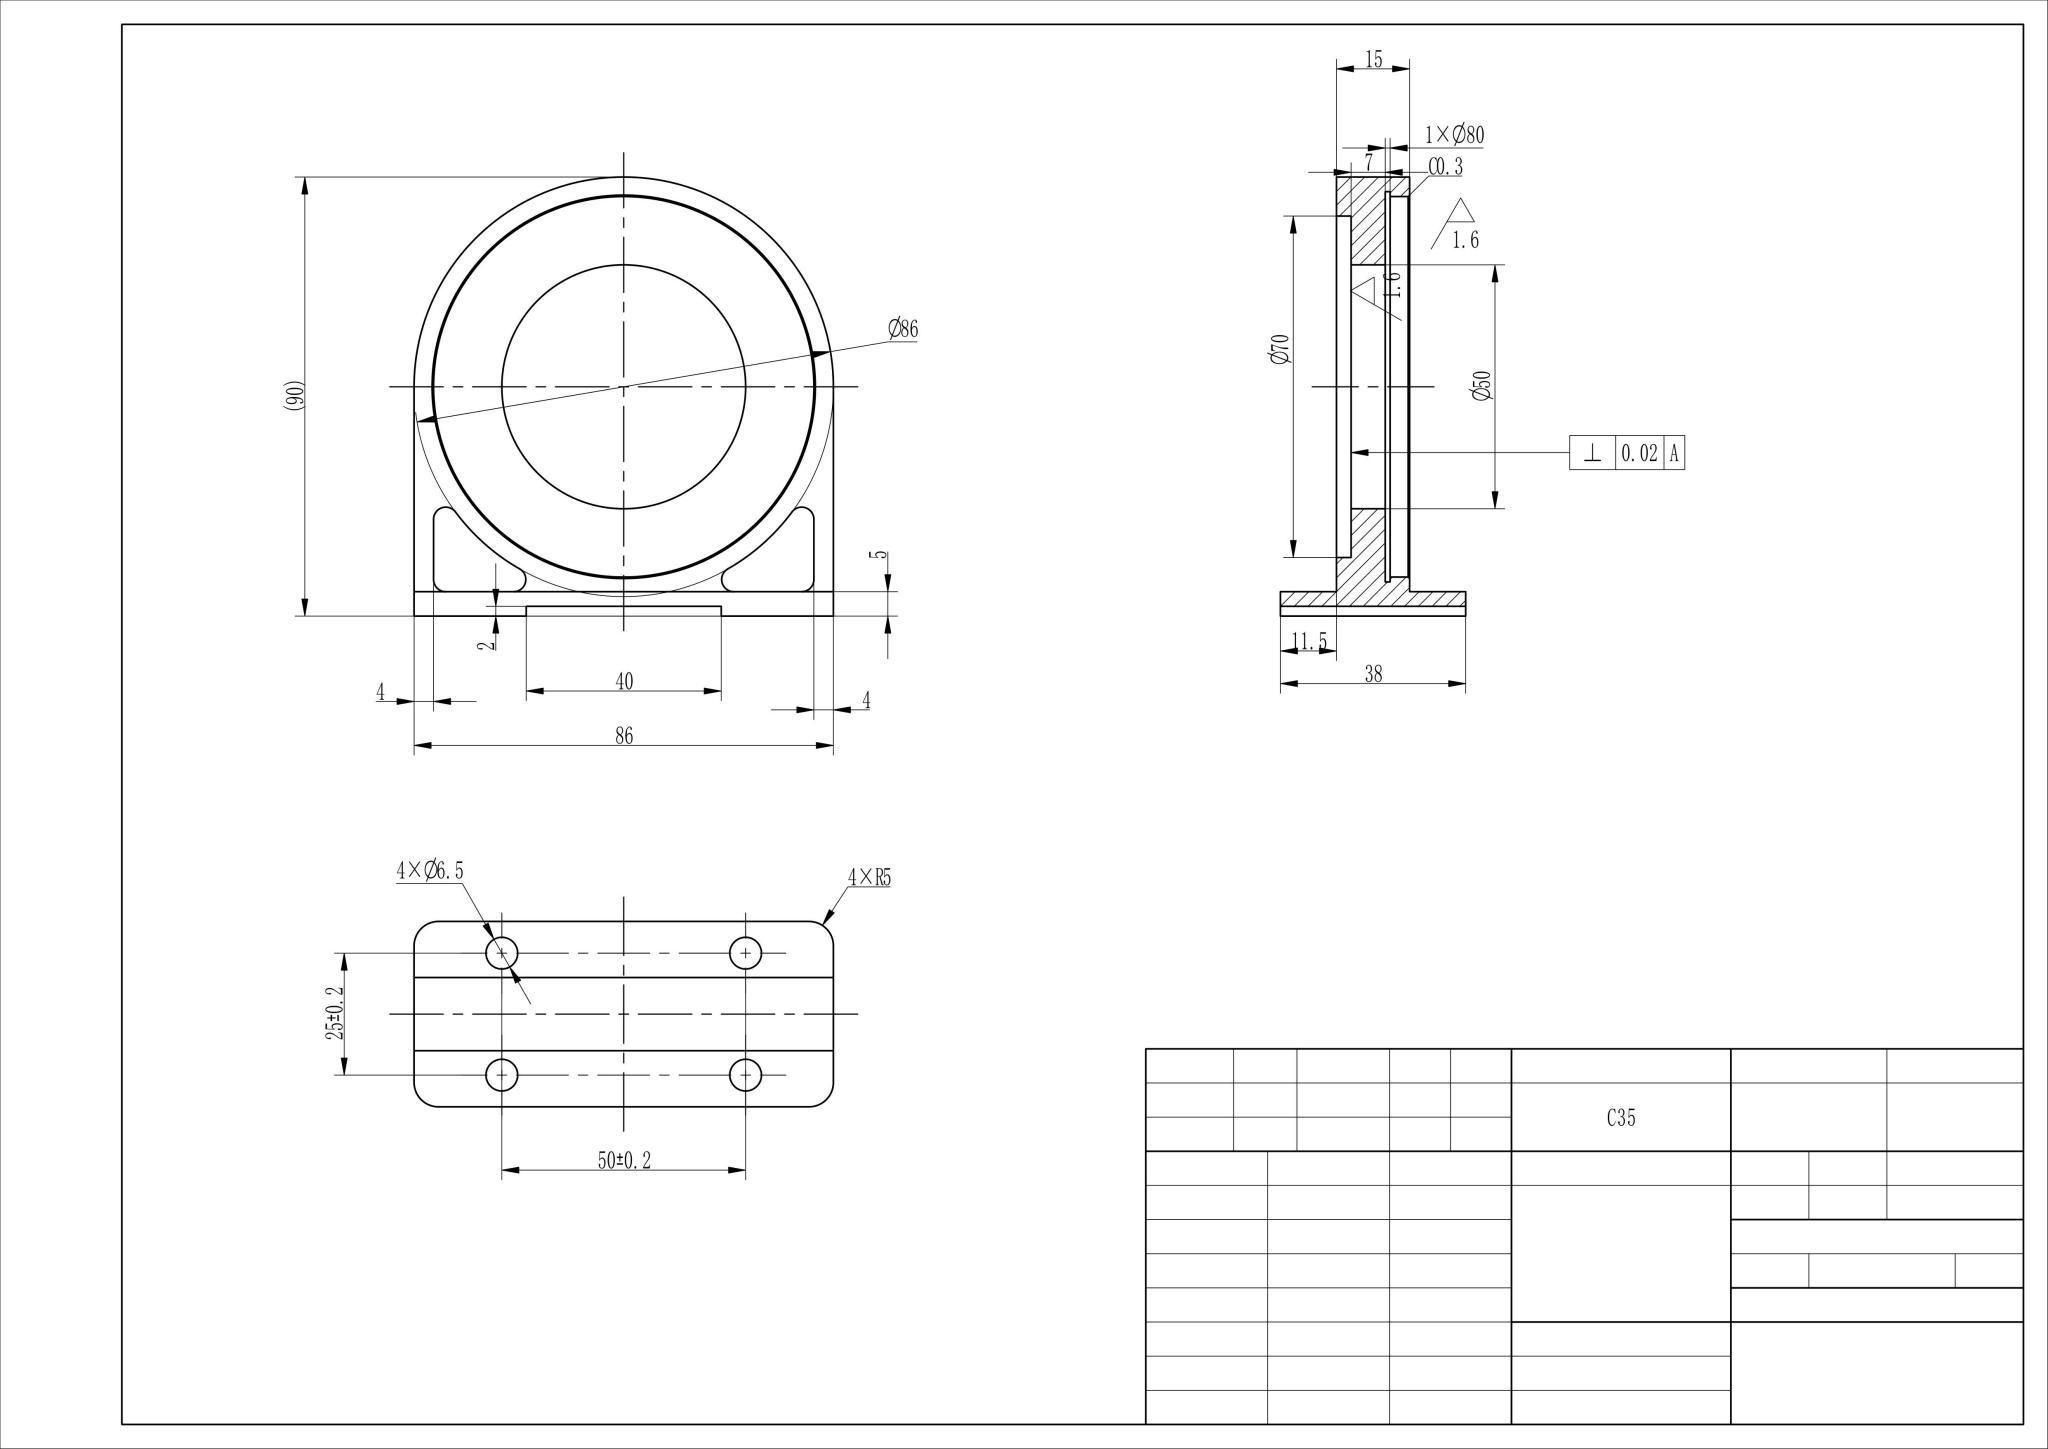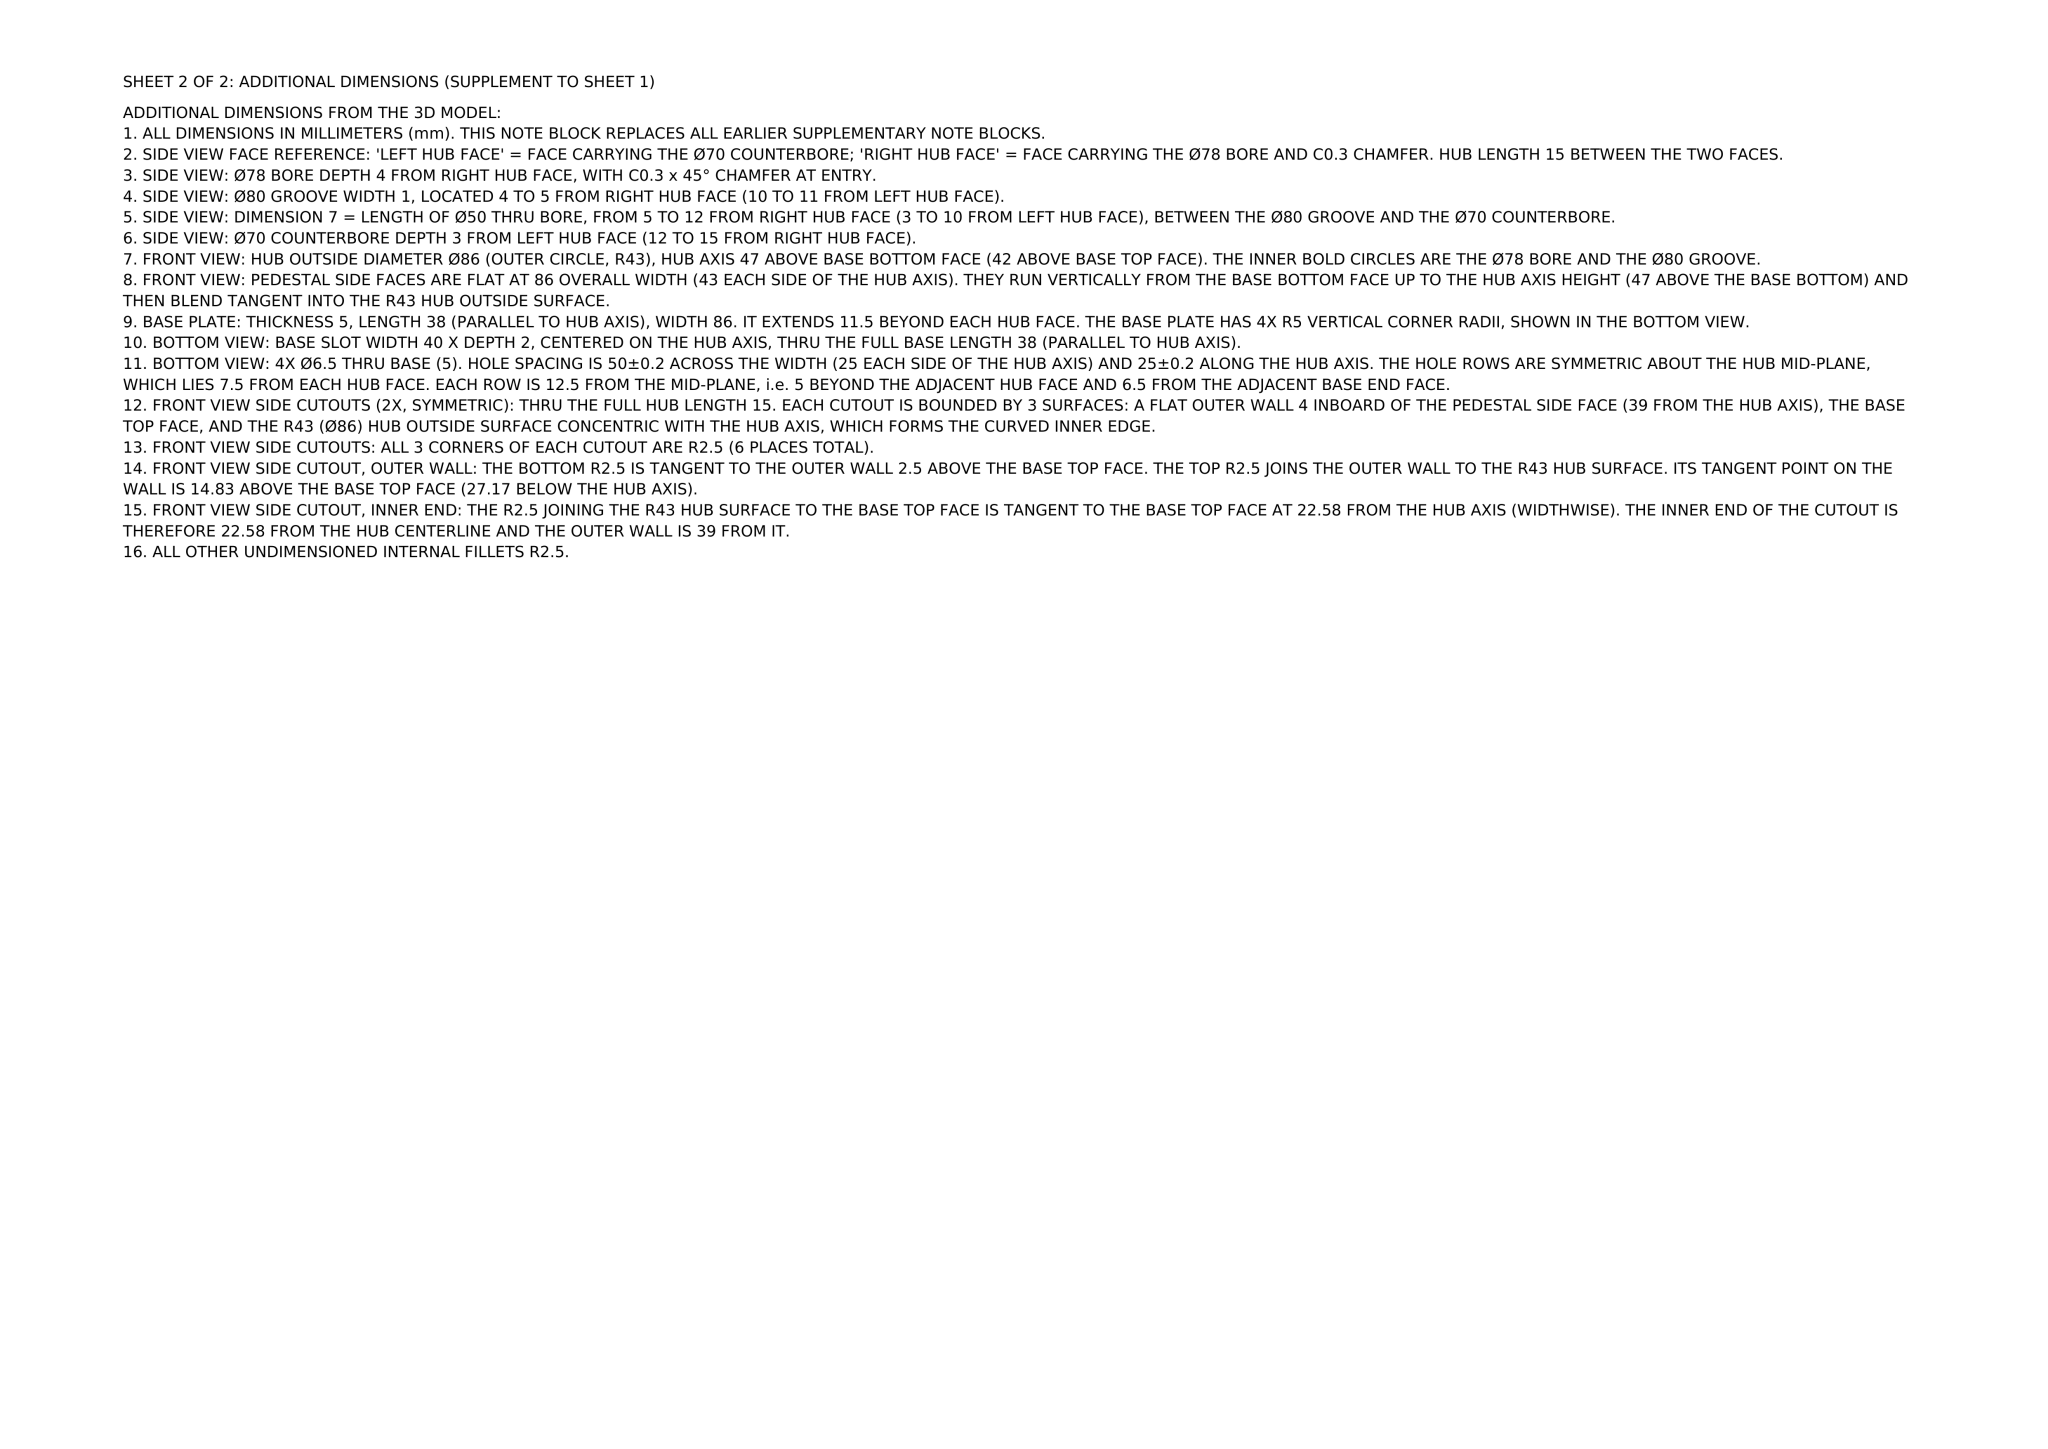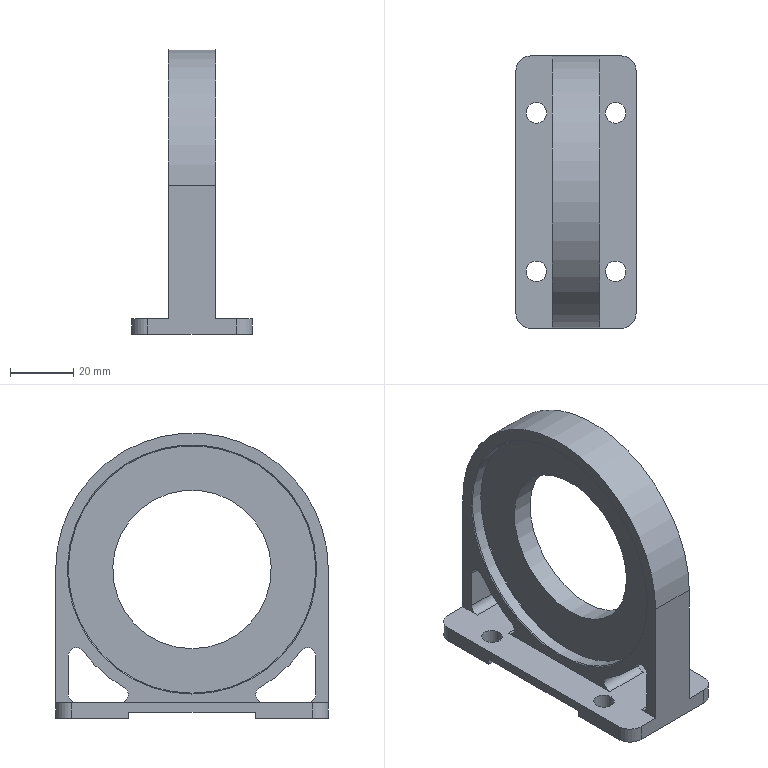Part | NX | mm | 1 solid | 39 faces | box 38 x 86 x 90 mm | volume 54655 mm3 | cylinder 21 | plane 17 | cone 1 | commonest cylinder face diameters 5 x6 6.5 x4 10 x4 86 x3 70 x1 78 x1 50 x1 80 x1